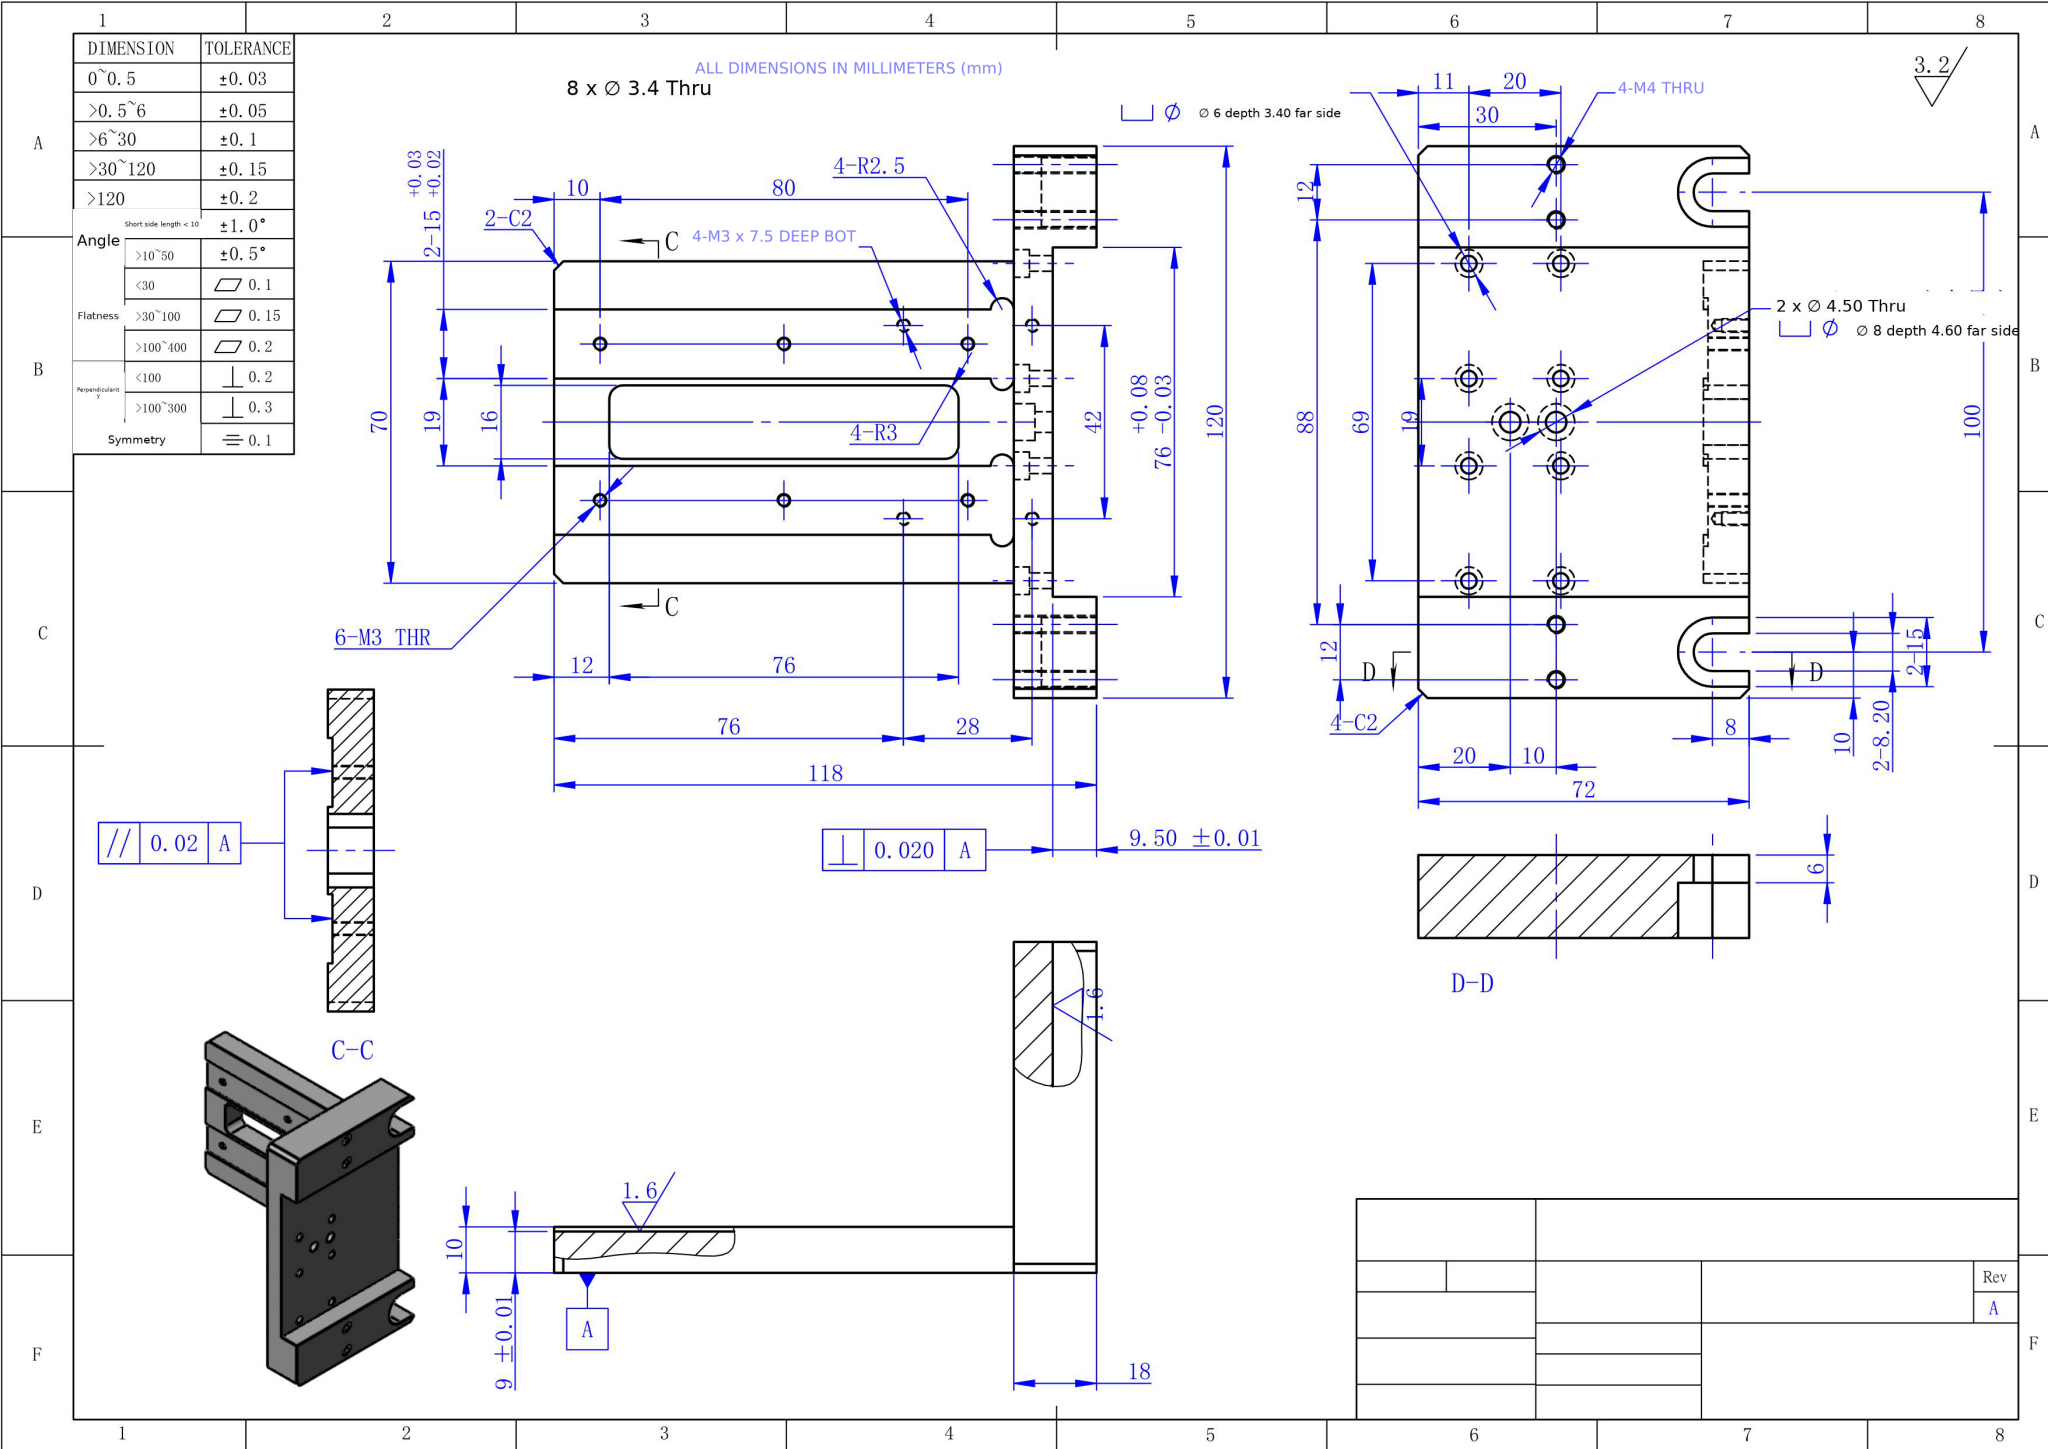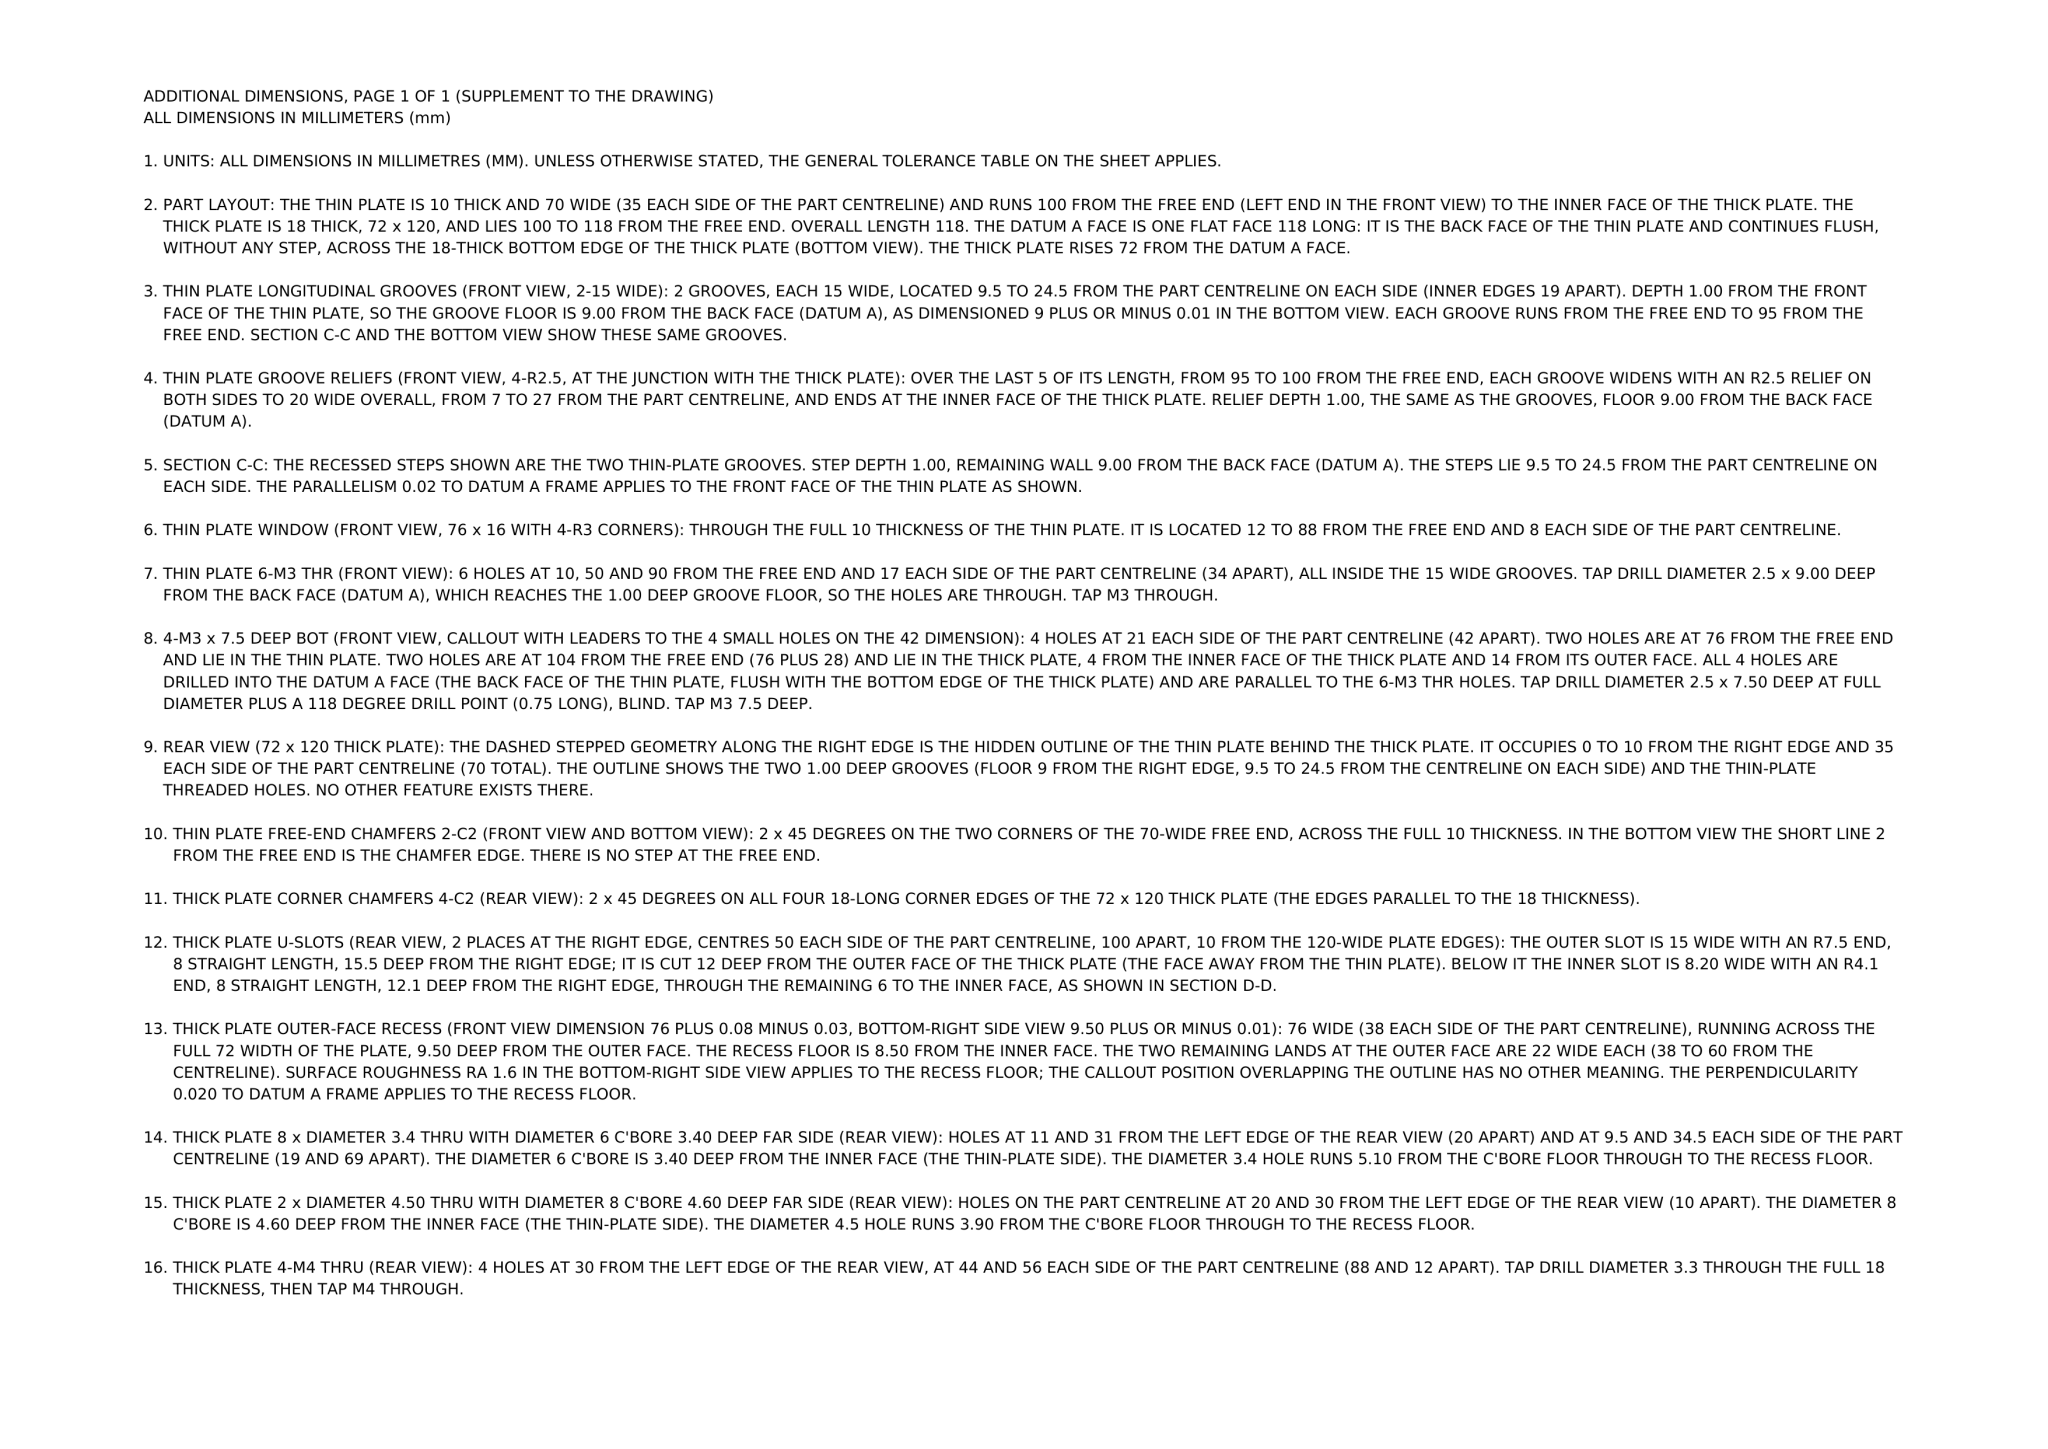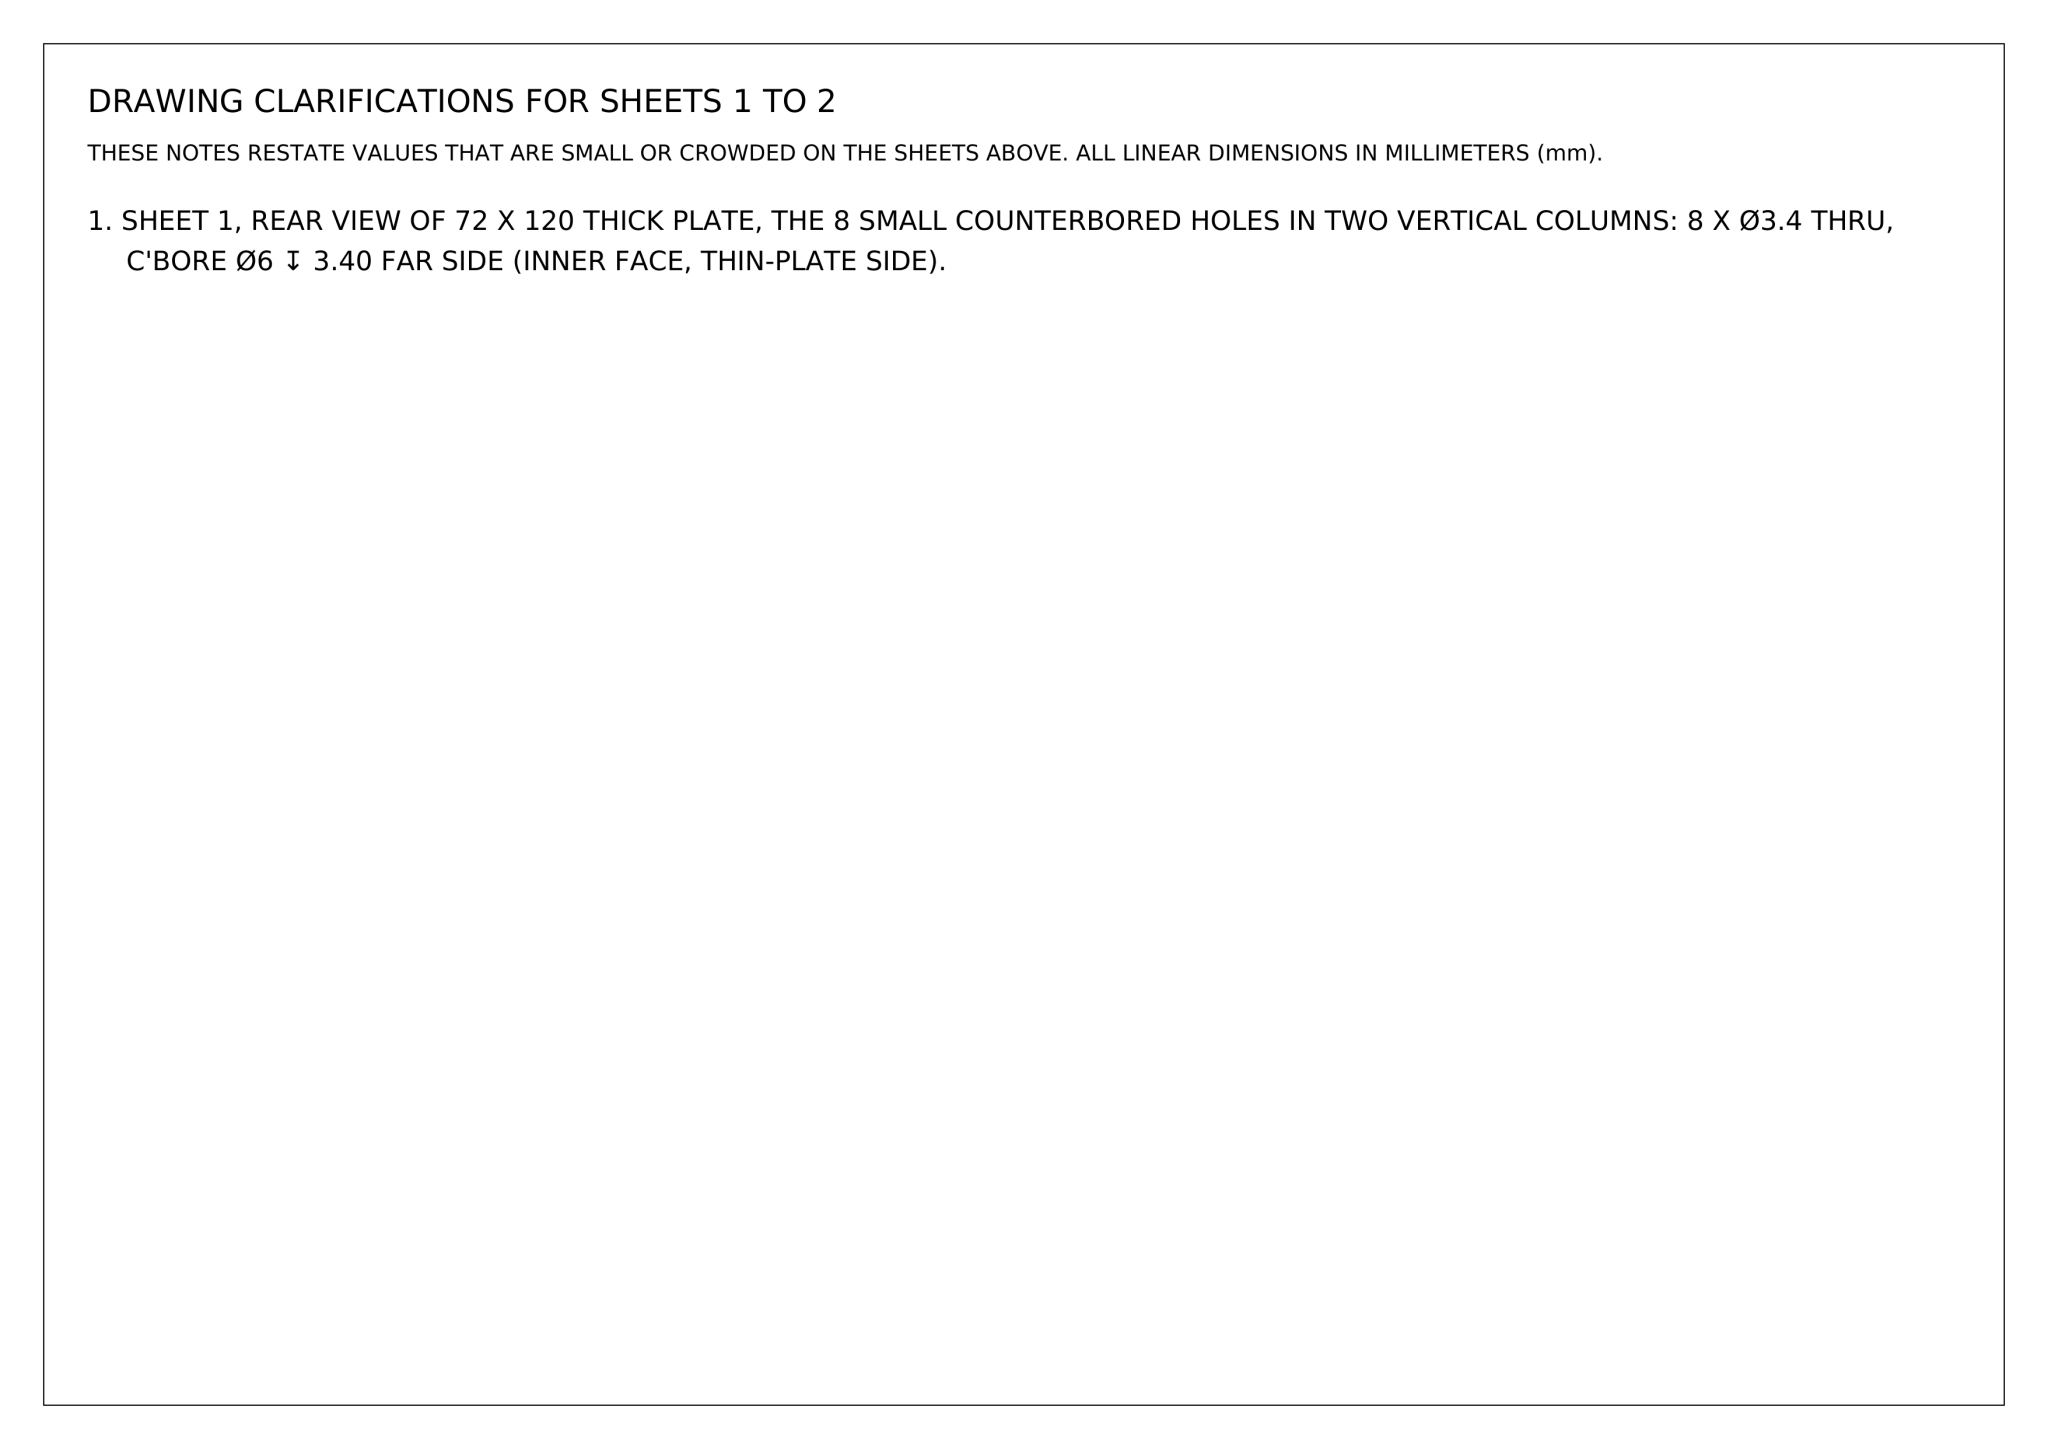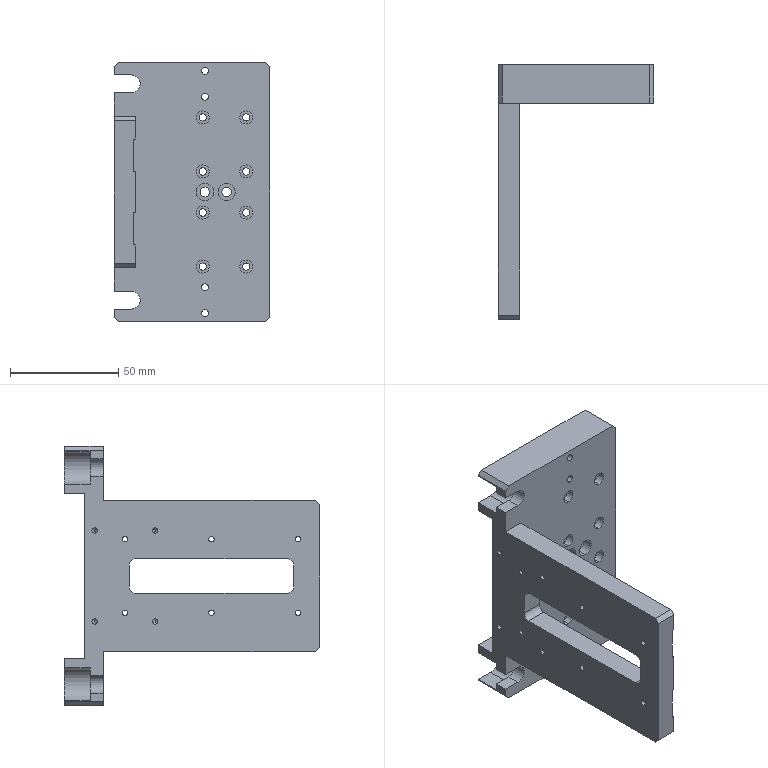Part | NX | mm | 1 solid | 142 faces | box 72 x 118 x 120 mm | volume 149366 mm3 | cylinder 80 | plane 54 | cone 8 | commonest cylinder face diameters 6 x20 2.5 x20 3.4 x16 3.3 x8 8 x4 4.5 x4 5 x4 8.2 x2